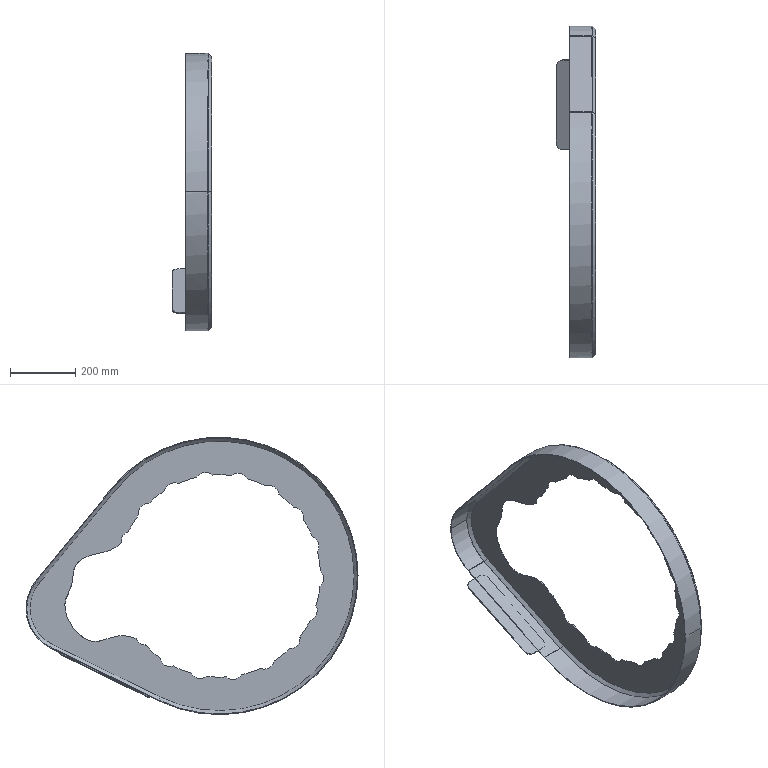Component | SolidWorks | ProtectiveCover-1 | 1 solid | 82 faces | volume 1121633 mm3 | cylinder 50 | plane 21 | cone 10 | spline 1 | commonest cylinder face diameters 61.909 x21 620 x15 40 x4 200 x3 270 x2 266 x2 846 x2 850 x1